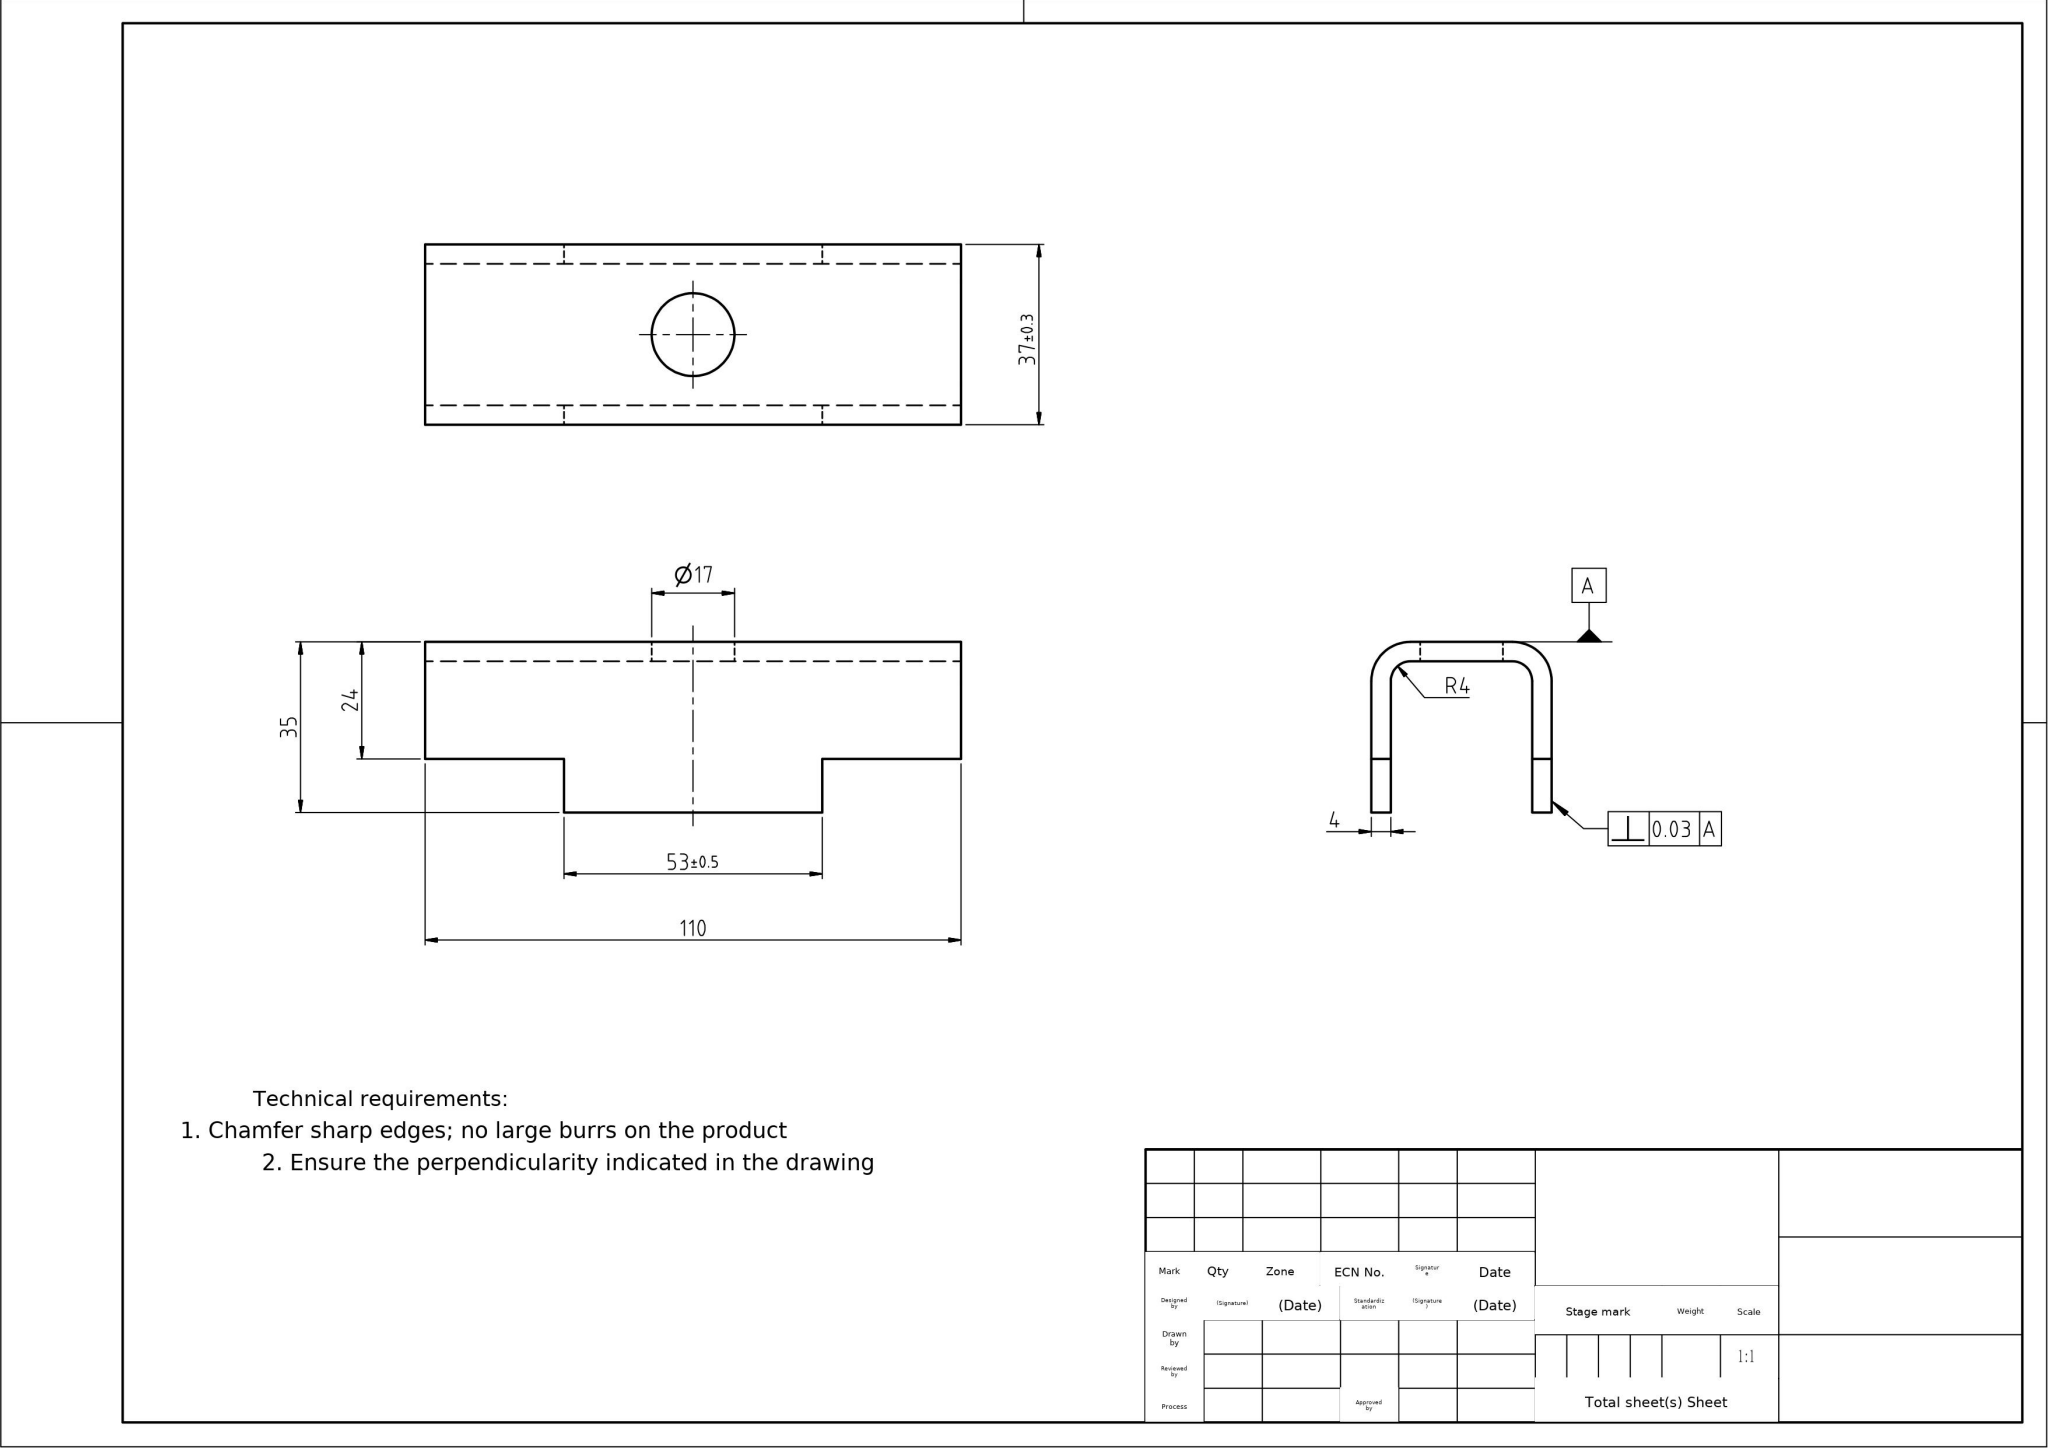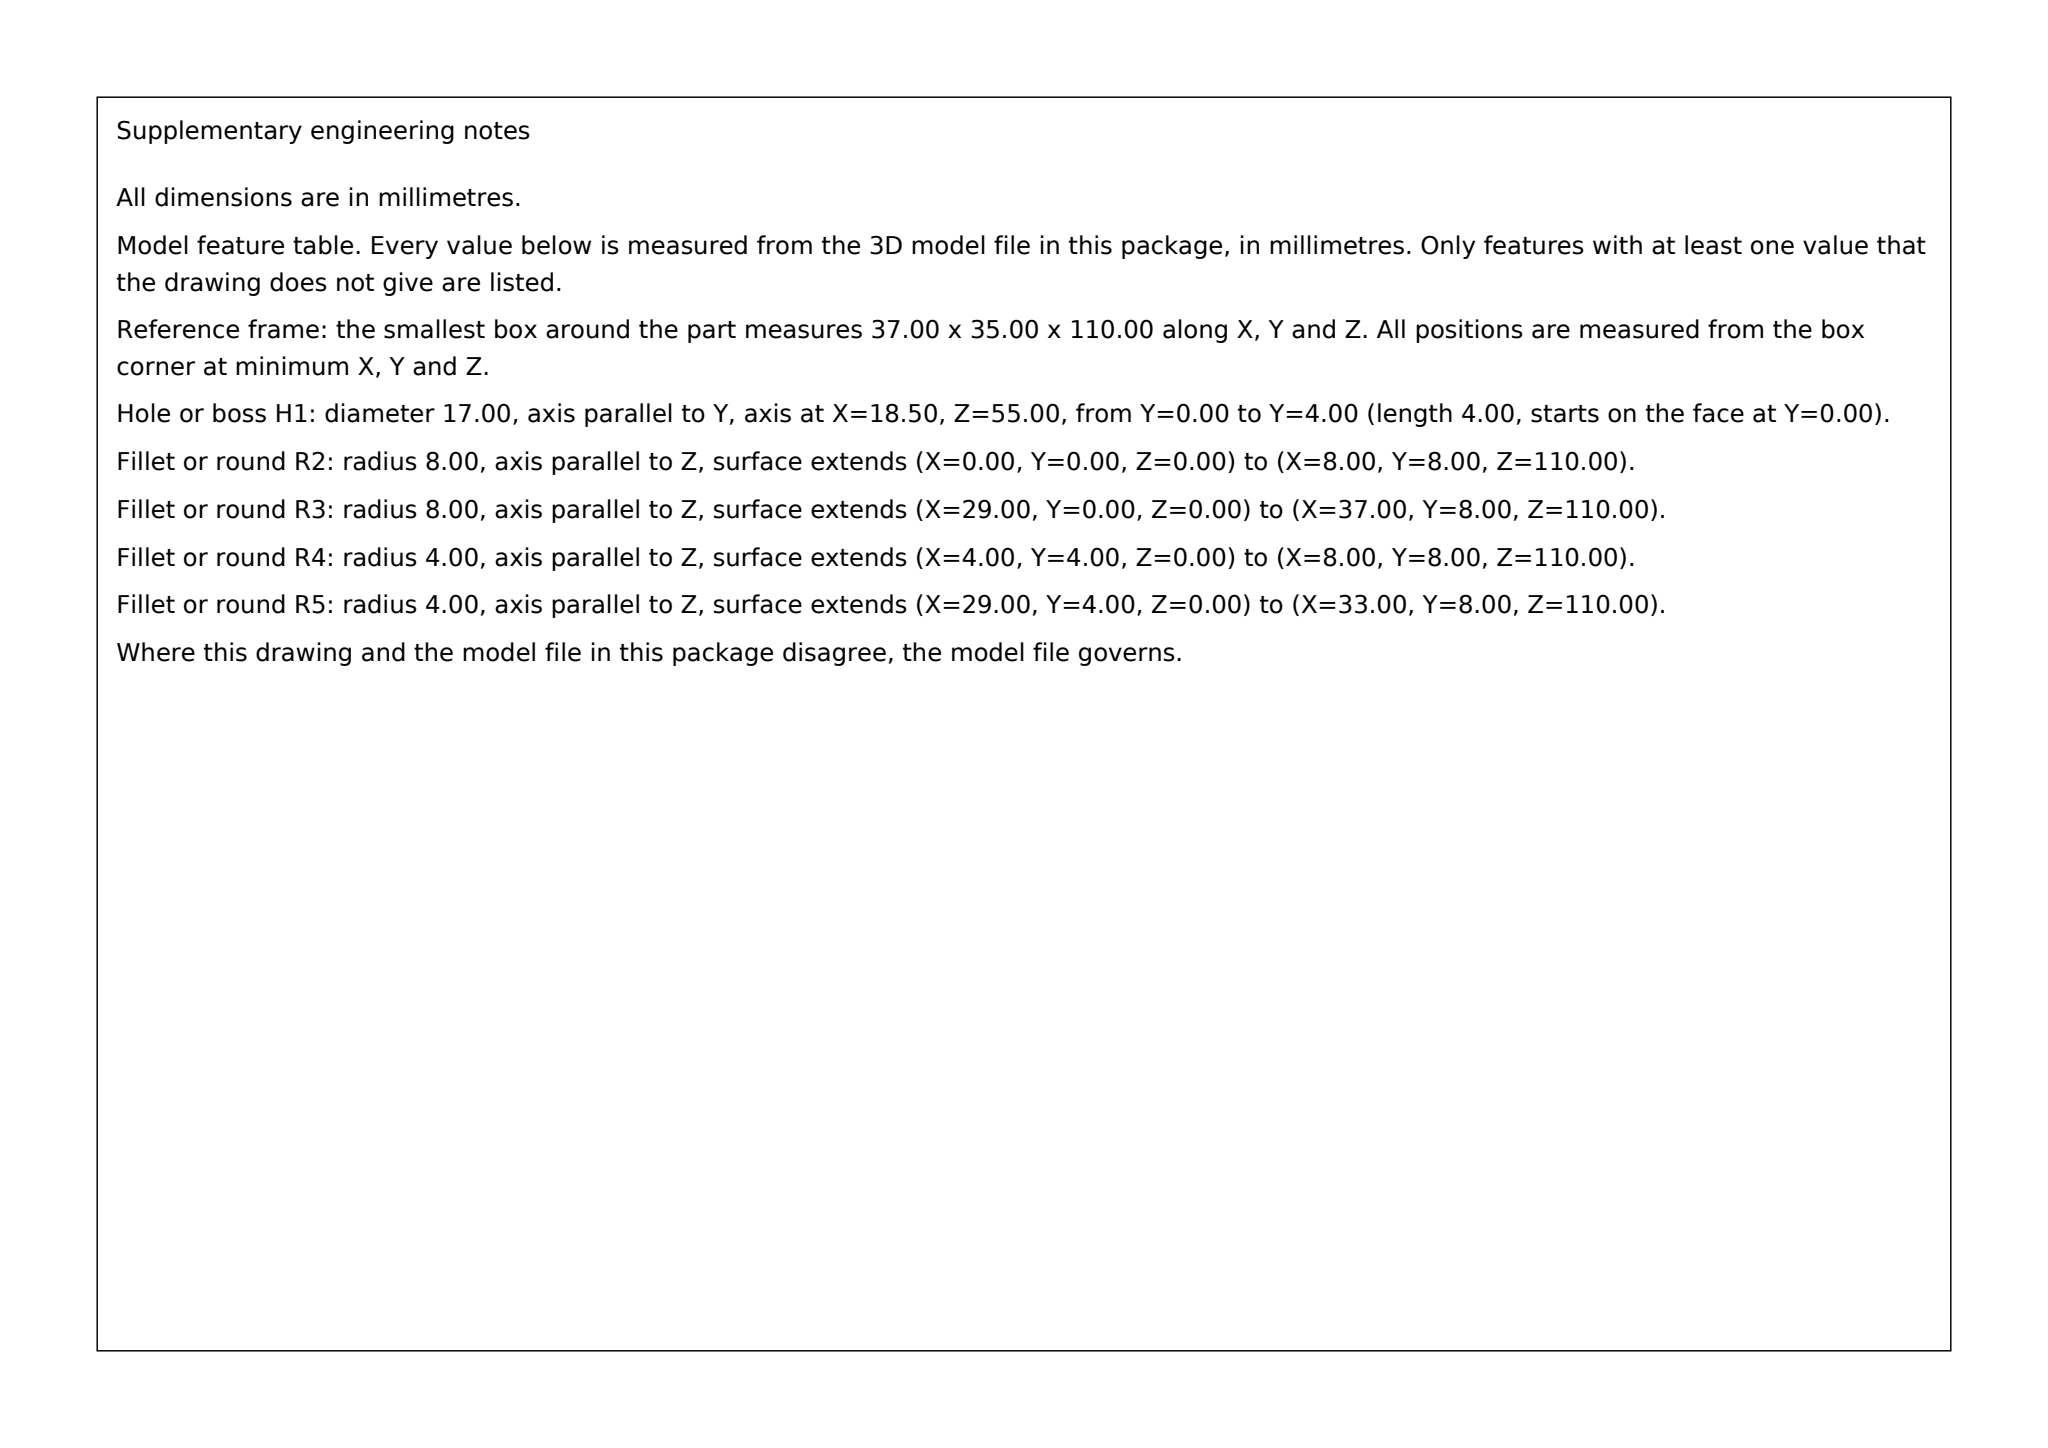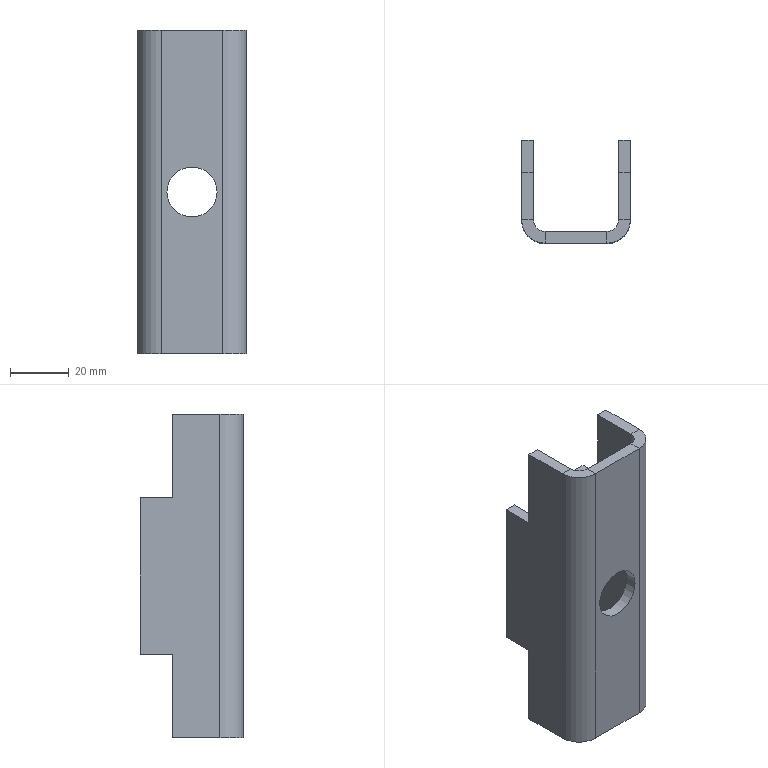Part | SolidWorks | mm | 1 solid | 32 faces | box 37 x 35 x 110 mm | volume 35370 mm3 | plane 26 | cylinder 6 | commonest cylinder face diameters 17 x2 16 x2 8 x2
STEP:
#1=CARTESIAN_POINT('',(-8.5,0.,-0.));
#2=VERTEX_POINT('',#1);
#3=CARTESIAN_POINT('',(8.5,0.,0.));
#4=VERTEX_POINT('',#3);
#5=CARTESIAN_POINT('',(0.,0.,0.));
#6=DIRECTION('',(0.,1.,0.));
#7=DIRECTION('',(1.,0.,0.));
#8=AXIS2_PLACEMENT_3D('',#5,#6,#7);
#9=CIRCLE('',#8,8.5);
#10=EDGE_CURVE('',#2,#4,#9,.T.);
#11=ORIENTED_EDGE('',*,*,#10,.F.);
#12=CARTESIAN_POINT('',(-8.5,4.,-0.));
#13=VERTEX_POINT('',#12);
#14=CARTESIAN_POINT('',(-8.5,0.,-0.));
#15=DIRECTION('',(0.,1.,0.));
#16=VECTOR('',#15,1000.);
#17=LINE('',#14,#16);
#18=EDGE_CURVE('',#2,#13,#17,.T.);
#19=ORIENTED_EDGE('',*,*,#18,.T.);
#20=CARTESIAN_POINT('',(8.5,4.,0.));
#21=VERTEX_POINT('',#20);
#22=CARTESIAN_POINT('',(0.,4.,0.));
#23=DIRECTION('',(0.,-1.,0.));
#24=DIRECTION('',(1.,0.,0.));
#25=AXIS2_PLACEMENT_3D('',#22,#23,#24);
#26=CIRCLE('',#25,8.5);
#27=EDGE_CURVE('',#21,#13,#26,.T.);
#28=ORIENTED_EDGE('',*,*,#27,.F.);
#29=CARTESIAN_POINT('',(8.5,0.,0.));
#30=DIRECTION('',(0.,1.,0.));
#31=VECTOR('',#30,1000.);
#32=LINE('',#29,#31);
#33=EDGE_CURVE('',#4,#21,#32,.T.);
#34=ORIENTED_EDGE('',*,*,#33,.F.);
#35=EDGE_LOOP('',(#11,#19,#28,#34));
#36=FACE_OUTER_BOUND('',#35,.T.);
#37=CARTESIAN_POINT('',(0.,0.,0.));
#38=DIRECTION('',(0.,1.,0.));
#39=DIRECTION('',(1.,0.,0.));
#40=AXIS2_PLACEMENT_3D('',#37,#38,#39);
#41=CYLINDRICAL_SURFACE('',#40,8.5);
#42=ADVANCED_FACE('',(#36),#41,.F.);
#43=CARTESIAN_POINT('',(18.5,35.,-26.5));
#44=VERTEX_POINT('',#43);
#45=CARTESIAN_POINT('',(14.5,35.,-26.5));
#46=VERTEX_POINT('',#45);
#47=CARTESIAN_POINT('',(16.5,35.,-26.5));
#48=DIRECTION('',(-1.,0.,-0.));
#49=VECTOR('',#48,1000.);
#50=LINE('',#47,#49);
#51=EDGE_CURVE('',#44,#46,#50,.T.);
#52=ORIENTED_EDGE('',*,*,#51,.F.);
#53=CARTESIAN_POINT('',(18.5,24.,-26.5));
#54=VERTEX_POINT('',#53);
#55=CARTESIAN_POINT('',(18.5,20.488,-26.5));
#56=DIRECTION('',(0.,1.,0.));
#57=VECTOR('',#56,1000.);
#58=LINE('',#55,#57);
#59=EDGE_CURVE('',#54,#44,#58,.T.);
#60=ORIENTED_EDGE('',*,*,#59,.F.);
#61=CARTESIAN_POINT('',(14.5,24.,-26.5));
#62=VERTEX_POINT('',#61);
#63=CARTESIAN_POINT('',(18.5,24.,-26.5));
#64=DIRECTION('',(-1.,0.,0.));
#65=VECTOR('',#64,1000.);
#66=LINE('',#63,#65);
#67=EDGE_CURVE('',#54,#62,#66,.T.);
#68=ORIENTED_EDGE('',*,*,#67,.T.);
#69=CARTESIAN_POINT('',(14.5,20.488,-26.5));
#70=DIRECTION('',(-0.,-1.,-0.));
#71=VECTOR('',#70,1000.);
#72=LINE('',#69,#71);
#73=EDGE_CURVE('',#46,#62,#72,.T.);
#74=ORIENTED_EDGE('',*,*,#73,.F.);
#75=EDGE_LOOP('',(#52,#60,#68,#74));
#76=FACE_OUTER_BOUND('',#75,.T.);
#77=CARTESIAN_POINT('',(18.5,24.,-26.5));
#78=DIRECTION('',(0.,-0.,1.));
#79=DIRECTION('',(1.,0.,0.));
#80=AXIS2_PLACEMENT_3D('',#77,#78,#79);
#81=PLANE('',#80);
#82=ADVANCED_FACE('',(#76),#81,.F.);
#83=CARTESIAN_POINT('',(14.5,24.,-55.));
#84=VERTEX_POINT('',#83);
#85=CARTESIAN_POINT('',(14.5,24.,-33.902));
#86=DIRECTION('',(0.,0.,-1.));
#87=VECTOR('',#86,1000.);
#88=LINE('',#85,#87);
#89=EDGE_CURVE('',#62,#84,#88,.T.);
#90=ORIENTED_EDGE('',*,*,#89,.F.);
#91=ORIENTED_EDGE('',*,*,#67,.F.);
#92=CARTESIAN_POINT('',(18.5,24.,-55.));
#93=VERTEX_POINT('',#92);
#94=CARTESIAN_POINT('',(18.5,24.,-33.902));
#95=DIRECTION('',(0.,-0.,1.));
#96=VECTOR('',#95,1000.);
#97=LINE('',#94,#96);
#98=EDGE_CURVE('',#93,#54,#97,.T.);
#99=ORIENTED_EDGE('',*,*,#98,.F.);
#100=CARTESIAN_POINT('',(16.5,24.,-55.));
#101=DIRECTION('',(1.,-0.,0.));
#102=VECTOR('',#101,1000.);
#103=LINE('',#100,#102);
#104=EDGE_CURVE('',#84,#93,#103,.T.);
#105=ORIENTED_EDGE('',*,*,#104,.F.);
#106=EDGE_LOOP('',(#90,#91,#99,#105));
#107=FACE_OUTER_BOUND('',#106,.T.);
#108=CARTESIAN_POINT('',(18.5,24.,-67.804));
#109=DIRECTION('',(-0.,-1.,-0.));
#110=DIRECTION('',(-1.,0.,0.));
#111=AXIS2_PLACEMENT_3D('',#108,#109,#110);
#112=PLANE('',#111);
#113=ADVANCED_FACE('',(#107),#112,.F.);
#114=CARTESIAN_POINT('',(-18.5,24.,-26.5));
#115=VERTEX_POINT('',#114);
#116=CARTESIAN_POINT('',(-18.5,24.,-55.));
#117=VERTEX_POINT('',#116);
#118=CARTESIAN_POINT('',(-18.5,24.,-33.902));
#119=DIRECTION('',(-0.,0.,-1.));
#120=VECTOR('',#119,1000.);
#121=LINE('',#118,#120);
#122=EDGE_CURVE('',#115,#117,#121,.T.);
#123=ORIENTED_EDGE('',*,*,#122,.F.);
#124=CARTESIAN_POINT('',(-14.5,24.,-26.5));
#125=VERTEX_POINT('',#124);
#126=CARTESIAN_POINT('',(18.5,24.,-26.5));
#127=DIRECTION('',(-1.,0.,0.));
#128=VECTOR('',#127,1000.);
#129=LINE('',#126,#128);
#130=EDGE_CURVE('',#125,#115,#129,.T.);
#131=ORIENTED_EDGE('',*,*,#130,.F.);
#132=CARTESIAN_POINT('',(-14.5,24.,-55.));
#133=VERTEX_POINT('',#132);
#134=CARTESIAN_POINT('',(-14.5,24.,-33.902));
#135=DIRECTION('',(0.,-0.,1.));
#136=VECTOR('',#135,1000.);
#137=LINE('',#134,#136);
#138=EDGE_CURVE('',#133,#125,#137,.T.);
#139=ORIENTED_EDGE('',*,*,#138,.F.);
#140=CARTESIAN_POINT('',(2.,24.,-55.));
#141=DIRECTION('',(1.,-0.,-0.));
#142=VECTOR('',#141,1000.);
#143=LINE('',#140,#142);
#144=EDGE_CURVE('',#117,#133,#143,.T.);
#145=ORIENTED_EDGE('',*,*,#144,.F.);
#146=EDGE_LOOP('',(#123,#131,#139,#145));
#147=FACE_OUTER_BOUND('',#146,.T.);
#148=CARTESIAN_POINT('',(18.5,24.,-67.804));
#149=DIRECTION('',(-0.,-1.,-0.));
#150=DIRECTION('',(-1.,0.,0.));
#151=AXIS2_PLACEMENT_3D('',#148,#149,#150);
#152=PLANE('',#151);
#153=ADVANCED_FACE('',(#147),#152,.F.);
#154=CARTESIAN_POINT('',(-18.5,35.,-26.5));
#155=VERTEX_POINT('',#154);
#156=CARTESIAN_POINT('',(-18.5,20.488,-26.5));
#157=DIRECTION('',(0.,-1.,-0.));
#158=VECTOR('',#157,1000.);
#159=LINE('',#156,#158);
#160=EDGE_CURVE('',#155,#115,#159,.T.);
#161=ORIENTED_EDGE('',*,*,#160,.F.);
#162=CARTESIAN_POINT('',(-14.5,35.,-26.5));
#163=VERTEX_POINT('',#162);
#164=CARTESIAN_POINT('',(2.,35.,-26.5));
#165=DIRECTION('',(-1.,-0.,-0.));
#166=VECTOR('',#165,1000.);
#167=LINE('',#164,#166);
#168=EDGE_CURVE('',#163,#155,#167,.T.);
#169=ORIENTED_EDGE('',*,*,#168,.F.);
#170=CARTESIAN_POINT('',(-14.5,20.488,-26.5));
#171=DIRECTION('',(-0.,1.,0.));
#172=VECTOR('',#171,1000.);
#173=LINE('',#170,#172);
#174=EDGE_CURVE('',#125,#163,#173,.T.);
#175=ORIENTED_EDGE('',*,*,#174,.F.);
#176=ORIENTED_EDGE('',*,*,#130,.T.);
#177=EDGE_LOOP('',(#161,#169,#175,#176));
#178=FACE_OUTER_BOUND('',#177,.T.);
#179=CARTESIAN_POINT('',(18.5,24.,-26.5));
#180=DIRECTION('',(0.,-0.,1.));
#181=DIRECTION('',(1.,0.,0.));
#182=AXIS2_PLACEMENT_3D('',#179,#180,#181);
#183=PLANE('',#182);
#184=ADVANCED_FACE('',(#178),#183,.F.);
#185=CARTESIAN_POINT('',(-18.5,24.,26.5));
#186=VERTEX_POINT('',#185);
#187=CARTESIAN_POINT('',(-18.5,35.,26.5));
#188=VERTEX_POINT('',#187);
#189=CARTESIAN_POINT('',(-18.5,30.405,26.5));
#190=DIRECTION('',(-0.,1.,0.));
#191=VECTOR('',#190,1000.);
#192=LINE('',#189,#191);
#193=EDGE_CURVE('',#186,#188,#192,.T.);
#194=ORIENTED_EDGE('',*,*,#193,.F.);
#195=CARTESIAN_POINT('',(-14.5,24.,26.5));
#196=VERTEX_POINT('',#195);
#197=CARTESIAN_POINT('',(18.5,24.,26.5));
#198=DIRECTION('',(-1.,0.,0.));
#199=VECTOR('',#198,1000.);
#200=LINE('',#197,#199);
#201=EDGE_CURVE('',#196,#186,#200,.T.);
#202=ORIENTED_EDGE('',*,*,#201,.F.);
#203=CARTESIAN_POINT('',(-14.5,35.,26.5));
#204=VERTEX_POINT('',#203);
#205=CARTESIAN_POINT('',(-14.5,30.405,26.5));
#206=DIRECTION('',(0.,-1.,0.));
#207=VECTOR('',#206,1000.);
#208=LINE('',#205,#207);
#209=EDGE_CURVE('',#204,#196,#208,.T.);
#210=ORIENTED_EDGE('',*,*,#209,.F.);
#211=CARTESIAN_POINT('',(2.,35.,26.5));
#212=DIRECTION('',(1.,0.,0.));
#213=VECTOR('',#212,1000.);
#214=LINE('',#211,#213);
#215=EDGE_CURVE('',#188,#204,#214,.T.);
#216=ORIENTED_EDGE('',*,*,#215,.F.);
#217=EDGE_LOOP('',(#194,#202,#210,#216));
#218=FACE_OUTER_BOUND('',#217,.T.);
#219=CARTESIAN_POINT('',(18.5,43.834,26.5));
#220=DIRECTION('',(0.,0.,-1.));
#221=DIRECTION('',(0.,-1.,0.));
#222=AXIS2_PLACEMENT_3D('',#219,#220,#221);
#223=PLANE('',#222);
#224=ADVANCED_FACE('',(#218),#223,.F.);
#225=CARTESIAN_POINT('',(-18.5,24.,55.));
#226=VERTEX_POINT('',#225);
#227=CARTESIAN_POINT('',(-18.5,24.,13.25));
#228=DIRECTION('',(-0.,0.,-1.));
#229=VECTOR('',#228,1000.);
#230=LINE('',#227,#229);
#231=EDGE_CURVE('',#226,#186,#230,.T.);
#232=ORIENTED_EDGE('',*,*,#231,.F.);
#233=CARTESIAN_POINT('',(-14.5,24.,55.));
#234=VERTEX_POINT('',#233);
#235=CARTESIAN_POINT('',(2.,24.,55.));
#236=DIRECTION('',(-1.,0.,0.));
#237=VECTOR('',#236,1000.);
#238=LINE('',#235,#237);
#239=EDGE_CURVE('',#234,#226,#238,.T.);
#240=ORIENTED_EDGE('',*,*,#239,.F.);
#241=CARTESIAN_POINT('',(-14.5,24.,13.25));
#242=DIRECTION('',(0.,-0.,1.));
#243=VECTOR('',#242,1000.);
#244=LINE('',#241,#243);
#245=EDGE_CURVE('',#196,#234,#244,.T.);
#246=ORIENTED_EDGE('',*,*,#245,.F.);
#247=ORIENTED_EDGE('',*,*,#201,.T.);
#248=EDGE_LOOP('',(#232,#240,#246,#247));
#249=FACE_OUTER_BOUND('',#248,.T.);
#250=CARTESIAN_POINT('',(18.5,24.,26.5));
#251=DIRECTION('',(-0.,-1.,-0.));
#252=DIRECTION('',(-1.,0.,0.));
#253=AXIS2_PLACEMENT_3D('',#250,#251,#252);
#254=PLANE('',#253);
#255=ADVANCED_FACE('',(#249),#254,.F.);
#256=CARTESIAN_POINT('',(18.5,24.,55.));
#257=VERTEX_POINT('',#256);
#258=CARTESIAN_POINT('',(14.5,24.,55.));
#259=VERTEX_POINT('',#258);
#260=CARTESIAN_POINT('',(16.5,24.,55.));
#261=DIRECTION('',(-1.,0.,0.));
#262=VECTOR('',#261,1000.);
#263=LINE('',#260,#262);
#264=EDGE_CURVE('',#257,#259,#263,.T.);
#265=ORIENTED_EDGE('',*,*,#264,.F.);
#266=CARTESIAN_POINT('',(18.5,24.,26.5));
#267=VERTEX_POINT('',#266);
#268=CARTESIAN_POINT('',(18.5,24.,13.25));
#269=DIRECTION('',(0.,-0.,1.));
#270=VECTOR('',#269,1000.);
#271=LINE('',#268,#270);
#272=EDGE_CURVE('',#267,#257,#271,.T.);
#273=ORIENTED_EDGE('',*,*,#272,.F.);
#274=CARTESIAN_POINT('',(14.5,24.,26.5));
#275=VERTEX_POINT('',#274);
#276=CARTESIAN_POINT('',(18.5,24.,26.5));
#277=DIRECTION('',(-1.,0.,0.));
#278=VECTOR('',#277,1000.);
#279=LINE('',#276,#278);
#280=EDGE_CURVE('',#267,#275,#279,.T.);
#281=ORIENTED_EDGE('',*,*,#280,.T.);
#282=CARTESIAN_POINT('',(14.5,24.,13.25));
#283=DIRECTION('',(0.,0.,-1.));
#284=VECTOR('',#283,1000.);
#285=LINE('',#282,#284);
#286=EDGE_CURVE('',#259,#275,#285,.T.);
#287=ORIENTED_EDGE('',*,*,#286,.F.);
#288=EDGE_LOOP('',(#265,#273,#281,#287));
#289=FACE_OUTER_BOUND('',#288,.T.);
#290=CARTESIAN_POINT('',(18.5,24.,26.5));
#291=DIRECTION('',(-0.,-1.,-0.));
#292=DIRECTION('',(-1.,0.,0.));
#293=AXIS2_PLACEMENT_3D('',#290,#291,#292);
#294=PLANE('',#293);
#295=ADVANCED_FACE('',(#289),#294,.F.);
#296=CARTESIAN_POINT('',(14.5,35.,26.5));
#297=VERTEX_POINT('',#296);
#298=CARTESIAN_POINT('',(18.5,35.,26.5));
#299=VERTEX_POINT('',#298);
#300=CARTESIAN_POINT('',(16.5,35.,26.5));
#301=DIRECTION('',(1.,-0.,0.));
#302=VECTOR('',#301,1000.);
#303=LINE('',#300,#302);
#304=EDGE_CURVE('',#297,#299,#303,.T.);
#305=ORIENTED_EDGE('',*,*,#304,.F.);
#306=CARTESIAN_POINT('',(14.5,30.405,26.5));
#307=DIRECTION('',(0.,1.,0.));
#308=VECTOR('',#307,1000.);
#309=LINE('',#306,#308);
#310=EDGE_CURVE('',#275,#297,#309,.T.);
#311=ORIENTED_EDGE('',*,*,#310,.F.);
#312=ORIENTED_EDGE('',*,*,#280,.F.);
#313=CARTESIAN_POINT('',(18.5,30.405,26.5));
#314=DIRECTION('',(-0.,-1.,0.));
#315=VECTOR('',#314,1000.);
#316=LINE('',#313,#315);
#317=EDGE_CURVE('',#299,#267,#316,.T.);
#318=ORIENTED_EDGE('',*,*,#317,.F.);
#319=EDGE_LOOP('',(#305,#311,#312,#318));
#320=FACE_OUTER_BOUND('',#319,.T.);
#321=CARTESIAN_POINT('',(18.5,43.834,26.5));
#322=DIRECTION('',(0.,0.,-1.));
#323=DIRECTION('',(0.,-1.,0.));
#324=AXIS2_PLACEMENT_3D('',#321,#322,#323);
#325=PLANE('',#324);
#326=ADVANCED_FACE('',(#320),#325,.F.);
#327=ORIENTED_EDGE('',*,*,#144,.T.);
#328=CARTESIAN_POINT('',(-14.5,8.,-55.));
#329=VERTEX_POINT('',#328);
#330=CARTESIAN_POINT('',(-14.5,-1.048,-55.));
#331=DIRECTION('',(-0.,1.,-0.));
#332=VECTOR('',#331,1000.);
#333=LINE('',#330,#332);
#334=EDGE_CURVE('',#329,#133,#333,.T.);
#335=ORIENTED_EDGE('',*,*,#334,.F.);
#336=CARTESIAN_POINT('',(-18.5,8.,-55.));
#337=VERTEX_POINT('',#336);
#338=CARTESIAN_POINT('',(-15.38,8.,-55.));
#339=DIRECTION('',(-1.,-0.,0.));
#340=VECTOR('',#339,1000.);
#341=LINE('',#338,#340);
#342=EDGE_CURVE('',#329,#337,#341,.T.);
#343=ORIENTED_EDGE('',*,*,#342,.T.);
#344=CARTESIAN_POINT('',(-18.5,8.,-55.));
#345=DIRECTION('',(-0.,1.,0.));
#346=VECTOR('',#345,1000.);
#347=LINE('',#344,#346);
#348=EDGE_CURVE('',#337,#117,#347,.T.);
#349=ORIENTED_EDGE('',*,*,#348,.T.);
#350=EDGE_LOOP('',(#327,#335,#343,#349));
#351=FACE_OUTER_BOUND('',#350,.T.);
#352=CARTESIAN_POINT('',(-14.5,8.,-55.));
#353=DIRECTION('',(-0.,-0.,-1.));
#354=DIRECTION('',(-1.,0.,0.));
#355=AXIS2_PLACEMENT_3D('',#352,#353,#354);
#356=PLANE('',#355);
#357=ADVANCED_FACE('',(#351),#356,.T.);
#358=ORIENTED_EDGE('',*,*,#264,.T.);
#359=CARTESIAN_POINT('',(14.5,8.,55.));
#360=VERTEX_POINT('',#359);
#361=CARTESIAN_POINT('',(14.5,-1.048,55.));
#362=DIRECTION('',(0.,1.,0.));
#363=VECTOR('',#362,1000.);
#364=LINE('',#361,#363);
#365=EDGE_CURVE('',#360,#259,#364,.T.);
#366=ORIENTED_EDGE('',*,*,#365,.F.);
#367=CARTESIAN_POINT('',(18.5,8.,55.));
#368=VERTEX_POINT('',#367);
#369=CARTESIAN_POINT('',(15.38,8.,55.));
#370=DIRECTION('',(1.,-0.,0.));
#371=VECTOR('',#370,1000.);
#372=LINE('',#369,#371);
#373=EDGE_CURVE('',#360,#368,#372,.T.);
#374=ORIENTED_EDGE('',*,*,#373,.T.);
#375=CARTESIAN_POINT('',(18.5,8.,55.));
#376=DIRECTION('',(0.,1.,0.));
#377=VECTOR('',#376,1000.);
#378=LINE('',#375,#377);
#379=EDGE_CURVE('',#368,#257,#378,.T.);
#380=ORIENTED_EDGE('',*,*,#379,.T.);
#381=EDGE_LOOP('',(#358,#366,#374,#380));
#382=FACE_OUTER_BOUND('',#381,.T.);
#383=CARTESIAN_POINT('',(14.5,8.,55.));
#384=DIRECTION('',(0.,0.,1.));
#385=DIRECTION('',(1.,0.,0.));
#386=AXIS2_PLACEMENT_3D('',#383,#384,#385);
#387=PLANE('',#386);
#388=ADVANCED_FACE('',(#382),#387,.T.);
#389=ORIENTED_EDGE('',*,*,#51,.T.);
#390=CARTESIAN_POINT('',(14.5,35.,55.));
#391=DIRECTION('',(0.,0.,-1.));
#392=VECTOR('',#391,1000.);
#393=LINE('',#390,#392);
#394=EDGE_CURVE('',#297,#46,#393,.T.);
#395=ORIENTED_EDGE('',*,*,#394,.F.);
#396=ORIENTED_EDGE('',*,*,#304,.T.);
#397=CARTESIAN_POINT('',(18.5,35.,55.));
#398=DIRECTION('',(0.,0.,-1.));
#399=VECTOR('',#398,1000.);
#400=LINE('',#397,#399);
#401=EDGE_CURVE('',#299,#44,#400,.T.);
#402=ORIENTED_EDGE('',*,*,#401,.T.);
#403=EDGE_LOOP('',(#389,#395,#396,#402));
#404=FACE_OUTER_BOUND('',#403,.T.);
#405=CARTESIAN_POINT('',(14.5,35.,55.));
#406=DIRECTION('',(0.,1.,0.));
#407=DIRECTION('',(1.,0.,-0.));
#408=AXIS2_PLACEMENT_3D('',#405,#406,#407);
#409=PLANE('',#408);
#410=ADVANCED_FACE('',(#404),#409,.T.);
#411=ORIENTED_EDGE('',*,*,#73,.T.);
#412=ORIENTED_EDGE('',*,*,#89,.T.);
#413=CARTESIAN_POINT('',(14.5,8.,-55.));
#414=VERTEX_POINT('',#413);
#415=CARTESIAN_POINT('',(14.5,-1.048,-55.));
#416=DIRECTION('',(0.,1.,0.));
#417=VECTOR('',#416,1000.);
#418=LINE('',#415,#417);
#419=EDGE_CURVE('',#414,#84,#418,.T.);
#420=ORIENTED_EDGE('',*,*,#419,.F.);
#421=CARTESIAN_POINT('',(14.5,8.,-0.));
#422=DIRECTION('',(-0.,0.,1.));
#423=VECTOR('',#422,1000.);
#424=LINE('',#421,#423);
#425=EDGE_CURVE('',#414,#360,#424,.T.);
#426=ORIENTED_EDGE('',*,*,#425,.T.);
#427=ORIENTED_EDGE('',*,*,#365,.T.);
#428=ORIENTED_EDGE('',*,*,#286,.T.);
#429=ORIENTED_EDGE('',*,*,#310,.T.);
#430=ORIENTED_EDGE('',*,*,#394,.T.);
#431=EDGE_LOOP('',(#411,#412,#420,#426,#427,#428,#429,#430));
#432=FACE_OUTER_BOUND('',#431,.T.);
#433=CARTESIAN_POINT('',(14.5,16.976,-0.));
#434=DIRECTION('',(-1.,0.,-0.));
#435=DIRECTION('',(-0.,0.,1.));
#436=AXIS2_PLACEMENT_3D('',#433,#434,#435);
#437=PLANE('',#436);
#438=ADVANCED_FACE('',(#432),#437,.T.);
#439=ORIENTED_EDGE('',*,*,#138,.T.);
#440=ORIENTED_EDGE('',*,*,#174,.T.);
#441=CARTESIAN_POINT('',(-14.5,35.,-55.));
#442=DIRECTION('',(0.,-0.,1.));
#443=VECTOR('',#442,1000.);
#444=LINE('',#441,#443);
#445=EDGE_CURVE('',#163,#204,#444,.T.);
#446=ORIENTED_EDGE('',*,*,#445,.T.);
#447=ORIENTED_EDGE('',*,*,#209,.T.);
#448=ORIENTED_EDGE('',*,*,#245,.T.);
#449=CARTESIAN_POINT('',(-14.5,8.,55.));
#450=VERTEX_POINT('',#449);
#451=CARTESIAN_POINT('',(-14.5,-1.048,55.));
#452=DIRECTION('',(-0.,1.,-0.));
#453=VECTOR('',#452,1000.);
#454=LINE('',#451,#453);
#455=EDGE_CURVE('',#450,#234,#454,.T.);
#456=ORIENTED_EDGE('',*,*,#455,.F.);
#457=CARTESIAN_POINT('',(-14.5,8.,0.));
#458=DIRECTION('',(-0.,0.,-1.));
#459=VECTOR('',#458,1000.);
#460=LINE('',#457,#459);
#461=EDGE_CURVE('',#450,#329,#460,.T.);
#462=ORIENTED_EDGE('',*,*,#461,.T.);
#463=ORIENTED_EDGE('',*,*,#334,.T.);
#464=EDGE_LOOP('',(#439,#440,#446,#447,#448,#456,#462,#463));
#465=FACE_OUTER_BOUND('',#464,.T.);
#466=CARTESIAN_POINT('',(-14.5,16.976,-0.));
#467=DIRECTION('',(1.,-0.,-0.));
#468=DIRECTION('',(0.,1.,-0.));
#469=AXIS2_PLACEMENT_3D('',#466,#467,#468);
#470=PLANE('',#469);
#471=ADVANCED_FACE('',(#465),#470,.T.);
#472=ORIENTED_EDGE('',*,*,#18,.F.);
#473=CARTESIAN_POINT('',(0.,0.,0.));
#474=DIRECTION('',(0.,1.,0.));
#475=DIRECTION('',(1.,0.,0.));
#476=AXIS2_PLACEMENT_3D('',#473,#474,#475);
#477=CIRCLE('',#476,8.5);
#478=EDGE_CURVE('',#4,#2,#477,.T.);
#479=ORIENTED_EDGE('',*,*,#478,.F.);
#480=ORIENTED_EDGE('',*,*,#33,.T.);
#481=CARTESIAN_POINT('',(0.,4.,0.));
#482=DIRECTION('',(0.,-1.,0.));
#483=DIRECTION('',(1.,0.,0.));
#484=AXIS2_PLACEMENT_3D('',#481,#482,#483);
#485=CIRCLE('',#484,8.5);
#486=EDGE_CURVE('',#13,#21,#485,.T.);
#487=ORIENTED_EDGE('',*,*,#486,.F.);
#488=EDGE_LOOP('',(#472,#479,#480,#487));
#489=FACE_OUTER_BOUND('',#488,.T.);
#490=CARTESIAN_POINT('',(0.,0.,0.));
#491=DIRECTION('',(0.,1.,0.));
#492=DIRECTION('',(1.,0.,0.));
#493=AXIS2_PLACEMENT_3D('',#490,#491,#492);
#494=CYLINDRICAL_SURFACE('',#493,8.5);
#495=ADVANCED_FACE('',(#489),#494,.F.);
#496=CARTESIAN_POINT('',(-18.5,8.,55.));
#497=VERTEX_POINT('',#496);
#498=CARTESIAN_POINT('',(-18.5,8.,0.));
#499=DIRECTION('',(0.,0.,1.));
#500=VECTOR('',#499,1000.);
#501=LINE('',#498,#500);
#502=EDGE_CURVE('',#337,#497,#501,.T.);
#503=ORIENTED_EDGE('',*,*,#502,.F.);
#504=CARTESIAN_POINT('',(-10.5,-0.,-55.));
#505=VERTEX_POINT('',#504);
#506=CARTESIAN_POINT('',(-10.5,8.,-55.));
#507=DIRECTION('',(-0.,0.,-1.));
#508=DIRECTION('',(-0.,-1.,0.));
#509=AXIS2_PLACEMENT_3D('',#506,#507,#508);
#510=CIRCLE('',#509,8.);
#511=EDGE_CURVE('',#505,#337,#510,.T.);
#512=ORIENTED_EDGE('',*,*,#511,.F.);
#513=CARTESIAN_POINT('',(-10.5,-0.,55.));
#514=VERTEX_POINT('',#513);
#515=CARTESIAN_POINT('',(-10.5,0.,27.5));
#516=DIRECTION('',(-0.,0.,-1.));
#517=VECTOR('',#516,1000.);
#518=LINE('',#515,#517);
#519=EDGE_CURVE('',#514,#505,#518,.T.);
#520=ORIENTED_EDGE('',*,*,#519,.F.);
#521=CARTESIAN_POINT('',(-10.5,8.,55.));
#522=DIRECTION('',(0.,0.,1.));
#523=DIRECTION('',(-1.,0.,0.));
#524=AXIS2_PLACEMENT_3D('',#521,#522,#523);
#525=CIRCLE('',#524,8.);
#526=EDGE_CURVE('',#497,#514,#525,.T.);
#527=ORIENTED_EDGE('',*,*,#526,.F.);
#528=EDGE_LOOP('',(#503,#512,#520,#527));
#529=FACE_OUTER_BOUND('',#528,.T.);
#530=CARTESIAN_POINT('',(-10.5,8.,0.));
#531=DIRECTION('',(-0.,0.,-1.));
#532=DIRECTION('',(0.,-1.,0.));
#533=AXIS2_PLACEMENT_3D('',#530,#531,#532);
#534=CYLINDRICAL_SURFACE('',#533,8.);
#535=ADVANCED_FACE('',(#529),#534,.T.);
#536=ORIENTED_EDGE('',*,*,#239,.T.);
#537=CARTESIAN_POINT('',(-18.5,-1.048,55.));
#538=DIRECTION('',(0.,-1.,0.));
#539=VECTOR('',#538,1000.);
#540=LINE('',#537,#539);
#541=EDGE_CURVE('',#226,#497,#540,.T.);
#542=ORIENTED_EDGE('',*,*,#541,.T.);
#543=CARTESIAN_POINT('',(-15.38,8.,55.));
#544=DIRECTION('',(1.,0.,-0.));
#545=VECTOR('',#544,1000.);
#546=LINE('',#543,#545);
#547=EDGE_CURVE('',#497,#450,#546,.T.);
#548=ORIENTED_EDGE('',*,*,#547,.T.);
#549=ORIENTED_EDGE('',*,*,#455,.T.);
#550=EDGE_LOOP('',(#536,#542,#548,#549));
#551=FACE_OUTER_BOUND('',#550,.T.);
#552=CARTESIAN_POINT('',(-14.5,8.,55.));
#553=DIRECTION('',(0.,0.,1.));
#554=DIRECTION('',(1.,-0.,0.));
#555=AXIS2_PLACEMENT_3D('',#552,#553,#554);
#556=PLANE('',#555);
#557=ADVANCED_FACE('',(#551),#556,.T.);
#558=ORIENTED_EDGE('',*,*,#342,.F.);
#559=CARTESIAN_POINT('',(-10.5,4.,-55.));
#560=VERTEX_POINT('',#559);
#561=CARTESIAN_POINT('',(-10.5,8.,-55.));
#562=DIRECTION('',(-0.,0.,-1.));
#563=DIRECTION('',(0.,-1.,0.));
#564=AXIS2_PLACEMENT_3D('',#561,#562,#563);
#565=CIRCLE('',#564,4.);
#566=EDGE_CURVE('',#560,#329,#565,.T.);
#567=ORIENTED_EDGE('',*,*,#566,.F.);
#568=CARTESIAN_POINT('',(-10.5,2.,-55.));
#569=DIRECTION('',(0.,1.,0.));
#570=VECTOR('',#569,1000.);
#571=LINE('',#568,#570);
#572=EDGE_CURVE('',#505,#560,#571,.T.);
#573=ORIENTED_EDGE('',*,*,#572,.F.);
#574=ORIENTED_EDGE('',*,*,#511,.T.);
#575=EDGE_LOOP('',(#558,#567,#573,#574));
#576=FACE_OUTER_BOUND('',#575,.T.);
#577=CARTESIAN_POINT('',(-14.5,8.,-55.));
#578=DIRECTION('',(-0.,0.,-1.));
#579=DIRECTION('',(-1.,0.,0.));
#580=AXIS2_PLACEMENT_3D('',#577,#578,#579);
#581=PLANE('',#580);
#582=ADVANCED_FACE('',(#576),#581,.T.);
#583=ORIENTED_EDGE('',*,*,#547,.F.);
#584=ORIENTED_EDGE('',*,*,#526,.T.);
#585=CARTESIAN_POINT('',(-10.5,4.,55.));
#586=VERTEX_POINT('',#585);
#587=CARTESIAN_POINT('',(-10.5,2.,55.));
#588=DIRECTION('',(0.,-1.,0.));
#589=VECTOR('',#588,1000.);
#590=LINE('',#587,#589);
#591=EDGE_CURVE('',#586,#514,#590,.T.);
#592=ORIENTED_EDGE('',*,*,#591,.F.);
#593=CARTESIAN_POINT('',(-10.5,8.,55.));
#594=DIRECTION('',(-0.,0.,-1.));
#595=DIRECTION('',(0.,-1.,0.));
#596=AXIS2_PLACEMENT_3D('',#593,#594,#595);
#597=CIRCLE('',#596,4.);
#598=EDGE_CURVE('',#586,#450,#597,.T.);
#599=ORIENTED_EDGE('',*,*,#598,.T.);
#600=EDGE_LOOP('',(#583,#584,#592,#599));
#601=FACE_OUTER_BOUND('',#600,.T.);
#602=CARTESIAN_POINT('',(-18.5,8.,55.));
#603=DIRECTION('',(0.,0.,1.));
#604=DIRECTION('',(1.,-0.,0.));
#605=AXIS2_PLACEMENT_3D('',#602,#603,#604);
#606=PLANE('',#605);
#607=ADVANCED_FACE('',(#601),#606,.T.);
#608=ORIENTED_EDGE('',*,*,#168,.T.);
#609=CARTESIAN_POINT('',(-18.5,35.,-55.));
#610=DIRECTION('',(0.,-0.,1.));
#611=VECTOR('',#610,1000.);
#612=LINE('',#609,#611);
#613=EDGE_CURVE('',#155,#188,#612,.T.);
#614=ORIENTED_EDGE('',*,*,#613,.T.);
#615=ORIENTED_EDGE('',*,*,#215,.T.);
#616=ORIENTED_EDGE('',*,*,#445,.F.);
#617=EDGE_LOOP('',(#608,#614,#615,#616));
#618=FACE_OUTER_BOUND('',#617,.T.);
#619=CARTESIAN_POINT('',(-14.5,35.,-55.));
#620=DIRECTION('',(-0.,1.,0.));
#621=DIRECTION('',(1.,0.,0.));
#622=AXIS2_PLACEMENT_3D('',#619,#620,#621);
#623=PLANE('',#622);
#624=ADVANCED_FACE('',(#618),#623,.T.);
#625=ORIENTED_EDGE('',*,*,#122,.T.);
#626=ORIENTED_EDGE('',*,*,#348,.F.);
#627=ORIENTED_EDGE('',*,*,#502,.T.);
#628=ORIENTED_EDGE('',*,*,#541,.F.);
#629=ORIENTED_EDGE('',*,*,#231,.T.);
#630=ORIENTED_EDGE('',*,*,#193,.T.);
#631=ORIENTED_EDGE('',*,*,#613,.F.);
#632=ORIENTED_EDGE('',*,*,#160,.T.);
#633=EDGE_LOOP('',(#625,#626,#627,#628,#629,#630,#631,#632));
#634=FACE_OUTER_BOUND('',#633,.T.);
#635=CARTESIAN_POINT('',(-18.5,16.976,0.));
#636=DIRECTION('',(1.,-0.,-0.));
#637=DIRECTION('',(0.,1.,-0.));
#638=AXIS2_PLACEMENT_3D('',#635,#636,#637);
#639=PLANE('',#638);
#640=ADVANCED_FACE('',(#634),#639,.F.);
#641=ORIENTED_EDGE('',*,*,#461,.F.);
#642=ORIENTED_EDGE('',*,*,#598,.F.);
#643=CARTESIAN_POINT('',(-10.5,4.,27.5));
#644=DIRECTION('',(0.,0.,1.));
#645=VECTOR('',#644,1000.);
#646=LINE('',#643,#645);
#647=EDGE_CURVE('',#560,#586,#646,.T.);
#648=ORIENTED_EDGE('',*,*,#647,.F.);
#649=ORIENTED_EDGE('',*,*,#566,.T.);
#650=EDGE_LOOP('',(#641,#642,#648,#649));
#651=FACE_OUTER_BOUND('',#650,.T.);
#652=CARTESIAN_POINT('',(-10.5,8.,0.));
#653=DIRECTION('',(-0.,0.,-1.));
#654=DIRECTION('',(0.,-1.,0.));
#655=AXIS2_PLACEMENT_3D('',#652,#653,#654);
#656=CYLINDRICAL_SURFACE('',#655,4.);
#657=ADVANCED_FACE('',(#651),#656,.F.);
#658=CARTESIAN_POINT('',(18.5,8.,-55.));
#659=VERTEX_POINT('',#658);
#660=CARTESIAN_POINT('',(18.5,8.,-0.));
#661=DIRECTION('',(-0.,0.,-1.));
#662=VECTOR('',#661,1000.);
#663=LINE('',#660,#662);
#664=EDGE_CURVE('',#368,#659,#663,.T.);
#665=ORIENTED_EDGE('',*,*,#664,.F.);
#666=CARTESIAN_POINT('',(10.5,-0.,55.));
#667=VERTEX_POINT('',#666);
#668=CARTESIAN_POINT('',(10.5,8.,55.));
#669=DIRECTION('',(0.,0.,1.));
#670=DIRECTION('',(0.,-1.,0.));
#671=AXIS2_PLACEMENT_3D('',#668,#669,#670);
#672=CIRCLE('',#671,8.);
#673=EDGE_CURVE('',#667,#368,#672,.T.);
#674=ORIENTED_EDGE('',*,*,#673,.F.);
#675=CARTESIAN_POINT('',(10.5,-0.,-55.));
#676=VERTEX_POINT('',#675);
#677=CARTESIAN_POINT('',(10.5,0.,-27.5));
#678=DIRECTION('',(0.,0.,1.));
#679=VECTOR('',#678,1000.);
#680=LINE('',#677,#679);
#681=EDGE_CURVE('',#676,#667,#680,.T.);
#682=ORIENTED_EDGE('',*,*,#681,.F.);
#683=CARTESIAN_POINT('',(10.5,8.,-55.));
#684=DIRECTION('',(0.,0.,-1.));
#685=DIRECTION('',(1.,-0.,0.));
#686=AXIS2_PLACEMENT_3D('',#683,#684,#685);
#687=CIRCLE('',#686,8.);
#688=EDGE_CURVE('',#659,#676,#687,.T.);
#689=ORIENTED_EDGE('',*,*,#688,.F.);
#690=EDGE_LOOP('',(#665,#674,#682,#689));
#691=FACE_OUTER_BOUND('',#690,.T.);
#692=CARTESIAN_POINT('',(10.5,8.,0.));
#693=DIRECTION('',(0.,0.,1.));
#694=DIRECTION('',(0.,-1.,0.));
#695=AXIS2_PLACEMENT_3D('',#692,#693,#694);
#696=CYLINDRICAL_SURFACE('',#695,8.);
#697=ADVANCED_FACE('',(#691),#696,.T.);
#698=ORIENTED_EDGE('',*,*,#104,.T.);
#699=CARTESIAN_POINT('',(18.5,-1.048,-55.));
#700=DIRECTION('',(-0.,-1.,0.));
#701=VECTOR('',#700,1000.);
#702=LINE('',#699,#701);
#703=EDGE_CURVE('',#93,#659,#702,.T.);
#704=ORIENTED_EDGE('',*,*,#703,.T.);
#705=CARTESIAN_POINT('',(15.38,8.,-55.));
#706=DIRECTION('',(-1.,0.,0.));
#707=VECTOR('',#706,1000.);
#708=LINE('',#705,#707);
#709=EDGE_CURVE('',#659,#414,#708,.T.);
#710=ORIENTED_EDGE('',*,*,#709,.T.);
#711=ORIENTED_EDGE('',*,*,#419,.T.);
#712=EDGE_LOOP('',(#698,#704,#710,#711));
#713=FACE_OUTER_BOUND('',#712,.T.);
#714=CARTESIAN_POINT('',(14.5,8.,-55.));
#715=DIRECTION('',(0.,0.,-1.));
#716=DIRECTION('',(0.,-1.,0.));
#717=AXIS2_PLACEMENT_3D('',#714,#715,#716);
#718=PLANE('',#717);
#719=ADVANCED_FACE('',(#713),#718,.T.);
#720=ORIENTED_EDGE('',*,*,#373,.F.);
#721=CARTESIAN_POINT('',(10.5,4.,55.));
#722=VERTEX_POINT('',#721);
#723=CARTESIAN_POINT('',(10.5,8.,55.));
#724=DIRECTION('',(0.,0.,1.));
#725=DIRECTION('',(0.,-1.,0.));
#726=AXIS2_PLACEMENT_3D('',#723,#724,#725);
#727=CIRCLE('',#726,4.);
#728=EDGE_CURVE('',#722,#360,#727,.T.);
#729=ORIENTED_EDGE('',*,*,#728,.F.);
#730=CARTESIAN_POINT('',(10.5,2.,55.));
#731=DIRECTION('',(0.,1.,0.));
#732=VECTOR('',#731,1000.);
#733=LINE('',#730,#732);
#734=EDGE_CURVE('',#667,#722,#733,.T.);
#735=ORIENTED_EDGE('',*,*,#734,.F.);
#736=ORIENTED_EDGE('',*,*,#673,.T.);
#737=EDGE_LOOP('',(#720,#729,#735,#736));
#738=FACE_OUTER_BOUND('',#737,.T.);
#739=CARTESIAN_POINT('',(14.5,8.,55.));
#740=DIRECTION('',(0.,0.,1.));
#741=DIRECTION('',(1.,0.,0.));
#742=AXIS2_PLACEMENT_3D('',#739,#740,#741);
#743=PLANE('',#742);
#744=ADVANCED_FACE('',(#738),#743,.T.);
#745=ORIENTED_EDGE('',*,*,#709,.F.);
#746=ORIENTED_EDGE('',*,*,#688,.T.);
#747=CARTESIAN_POINT('',(10.5,4.,-55.));
#748=VERTEX_POINT('',#747);
#749=CARTESIAN_POINT('',(10.5,2.,-55.));
#750=DIRECTION('',(0.,-1.,0.));
#751=VECTOR('',#750,1000.);
#752=LINE('',#749,#751);
#753=EDGE_CURVE('',#748,#676,#752,.T.);
#754=ORIENTED_EDGE('',*,*,#753,.F.);
#755=CARTESIAN_POINT('',(10.5,8.,-55.));
#756=DIRECTION('',(0.,0.,1.));
#757=DIRECTION('',(0.,-1.,0.));
#758=AXIS2_PLACEMENT_3D('',#755,#756,#757);
#759=CIRCLE('',#758,4.);
#760=EDGE_CURVE('',#748,#414,#759,.T.);
#761=ORIENTED_EDGE('',*,*,#760,.T.);
#762=EDGE_LOOP('',(#745,#746,#754,#761));
#763=FACE_OUTER_BOUND('',#762,.T.);
#764=CARTESIAN_POINT('',(18.5,8.,-55.));
#765=DIRECTION('',(0.,0.,-1.));
#766=DIRECTION('',(0.,-1.,0.));
#767=AXIS2_PLACEMENT_3D('',#764,#765,#766);
#768=PLANE('',#767);
#769=ADVANCED_FACE('',(#763),#768,.T.);
#770=ORIENTED_EDGE('',*,*,#59,.T.);
#771=ORIENTED_EDGE('',*,*,#401,.F.);
#772=ORIENTED_EDGE('',*,*,#317,.T.);
#773=ORIENTED_EDGE('',*,*,#272,.T.);
#774=ORIENTED_EDGE('',*,*,#379,.F.);
#775=ORIENTED_EDGE('',*,*,#664,.T.);
#776=ORIENTED_EDGE('',*,*,#703,.F.);
#777=ORIENTED_EDGE('',*,*,#98,.T.);
#778=EDGE_LOOP('',(#770,#771,#772,#773,#774,#775,#776,#777));
#779=FACE_OUTER_BOUND('',#778,.T.);
#780=CARTESIAN_POINT('',(18.5,16.976,-0.));
#781=DIRECTION('',(-1.,0.,0.));
#782=DIRECTION('',(0.,0.,1.));
#783=AXIS2_PLACEMENT_3D('',#780,#781,#782);
#784=PLANE('',#783);
#785=ADVANCED_FACE('',(#779),#784,.F.);
#786=ORIENTED_EDGE('',*,*,#425,.F.);
#787=ORIENTED_EDGE('',*,*,#760,.F.);
#788=CARTESIAN_POINT('',(10.5,4.,-27.5));
#789=DIRECTION('',(0.,0.,-1.));
#790=VECTOR('',#789,1000.);
#791=LINE('',#788,#790);
#792=EDGE_CURVE('',#722,#748,#791,.T.);
#793=ORIENTED_EDGE('',*,*,#792,.F.);
#794=ORIENTED_EDGE('',*,*,#728,.T.);
#795=EDGE_LOOP('',(#786,#787,#793,#794));
#796=FACE_OUTER_BOUND('',#795,.T.);
#797=CARTESIAN_POINT('',(10.5,8.,0.));
#798=DIRECTION('',(0.,0.,1.));
#799=DIRECTION('',(0.,-1.,0.));
#800=AXIS2_PLACEMENT_3D('',#797,#798,#799);
#801=CYLINDRICAL_SURFACE('',#800,4.);
#802=ADVANCED_FACE('',(#796),#801,.F.);
#803=ORIENTED_EDGE('',*,*,#591,.T.);
#804=CARTESIAN_POINT('',(-18.5,0.,55.));
#805=DIRECTION('',(1.,0.,-0.));
#806=VECTOR('',#805,1000.);
#807=LINE('',#804,#806);
#808=EDGE_CURVE('',#514,#667,#807,.T.);
#809=ORIENTED_EDGE('',*,*,#808,.T.);
#810=ORIENTED_EDGE('',*,*,#734,.T.);
#811=CARTESIAN_POINT('',(-18.5,4.,55.));
#812=DIRECTION('',(-1.,0.,0.));
#813=VECTOR('',#812,1000.);
#814=LINE('',#811,#813);
#815=EDGE_CURVE('',#722,#586,#814,.T.);
#816=ORIENTED_EDGE('',*,*,#815,.T.);
#817=EDGE_LOOP('',(#803,#809,#810,#816));
#818=FACE_OUTER_BOUND('',#817,.T.);
#819=CARTESIAN_POINT('',(18.5,0.,55.));
#820=DIRECTION('',(0.,0.,1.));
#821=DIRECTION('',(1.,-0.,0.));
#822=AXIS2_PLACEMENT_3D('',#819,#820,#821);
#823=PLANE('',#822);
#824=ADVANCED_FACE('',(#818),#823,.T.);
#825=ORIENTED_EDGE('',*,*,#519,.T.);
#826=CARTESIAN_POINT('',(18.5,0.,-55.));
#827=DIRECTION('',(-1.,0.,0.));
#828=VECTOR('',#827,1000.);
#829=LINE('',#826,#828);
#830=EDGE_CURVE('',#676,#505,#829,.T.);
#831=ORIENTED_EDGE('',*,*,#830,.F.);
#832=ORIENTED_EDGE('',*,*,#681,.T.);
#833=ORIENTED_EDGE('',*,*,#808,.F.);
#834=EDGE_LOOP('',(#825,#831,#832,#833));
#835=FACE_OUTER_BOUND('',#834,.T.);
#836=ORIENTED_EDGE('',*,*,#478,.T.);
#837=ORIENTED_EDGE('',*,*,#10,.T.);
#838=EDGE_LOOP('',(#836,#837));
#839=FACE_BOUND('',#838,.T.);
#840=CARTESIAN_POINT('',(0.,0.,-0.));
#841=DIRECTION('',(0.,1.,0.));
#842=DIRECTION('',(1.,0.,0.));
#843=AXIS2_PLACEMENT_3D('',#840,#841,#842);
#844=PLANE('',#843);
#845=ADVANCED_FACE('',(#835,#839),#844,.F.);
#846=ORIENTED_EDGE('',*,*,#572,.T.);
#847=CARTESIAN_POINT('',(18.5,4.,-55.));
#848=DIRECTION('',(1.,0.,0.));
#849=VECTOR('',#848,1000.);
#850=LINE('',#847,#849);
#851=EDGE_CURVE('',#560,#748,#850,.T.);
#852=ORIENTED_EDGE('',*,*,#851,.T.);
#853=ORIENTED_EDGE('',*,*,#753,.T.);
#854=ORIENTED_EDGE('',*,*,#830,.T.);
#855=EDGE_LOOP('',(#846,#852,#853,#854));
#856=FACE_OUTER_BOUND('',#855,.T.);
#857=CARTESIAN_POINT('',(-18.5,0.,-55.));
#858=DIRECTION('',(0.,0.,-1.));
#859=DIRECTION('',(0.,-1.,0.));
#860=AXIS2_PLACEMENT_3D('',#857,#858,#859);
#861=PLANE('',#860);
#862=ADVANCED_FACE('',(#856),#861,.T.);
#863=ORIENTED_EDGE('',*,*,#647,.T.);
#864=ORIENTED_EDGE('',*,*,#815,.F.);
#865=ORIENTED_EDGE('',*,*,#792,.T.);
#866=ORIENTED_EDGE('',*,*,#851,.F.);
#867=EDGE_LOOP('',(#863,#864,#865,#866));
#868=FACE_OUTER_BOUND('',#867,.T.);
#869=ORIENTED_EDGE('',*,*,#27,.T.);
#870=ORIENTED_EDGE('',*,*,#486,.T.);
#871=EDGE_LOOP('',(#869,#870));
#872=FACE_BOUND('',#871,.T.);
#873=CARTESIAN_POINT('',(0.,4.,-0.));
#874=DIRECTION('',(0.,1.,0.));
#875=DIRECTION('',(1.,0.,0.));
#876=AXIS2_PLACEMENT_3D('',#873,#874,#875);
#877=PLANE('',#876);
#878=ADVANCED_FACE('',(#868,#872),#877,.T.);
#879=CLOSED_SHELL('',(#42,#82,#113,#153,#184,#224,#255,#295,#326,#357,#388,#410,#438,#471,#495,#535,#557,#582,#607,#624,#640,#657,#697,#719,#744,#769,#785,#802,#824,#845,#862,#878));
#880=MANIFOLD_SOLID_BREP('',#879);
#881=CARTESIAN_POINT('',(0.,0.,0.));
#882=DIRECTION('',(0.,0.,1.));
#883=DIRECTION('',(1.,0.,0.));
#884=AXIS2_PLACEMENT_3D('',#881,#882,#883);
#885=(LENGTH_UNIT()NAMED_UNIT(*)SI_UNIT(.MILLI.,.METRE.));
#886=UNCERTAINTY_MEASURE_WITH_UNIT(LENGTH_MEASURE(0.00001),#885,'','');
#887=(NAMED_UNIT(*)PLANE_ANGLE_UNIT()SI_UNIT($,.RADIAN.));
#888=(NAMED_UNIT(*)SI_UNIT($,.STERADIAN.)SOLID_ANGLE_UNIT());
#889=(GEOMETRIC_REPRESENTATION_CONTEXT(3)GLOBAL_UNCERTAINTY_ASSIGNED_CONTEXT((#886))GLOBAL_UNIT_ASSIGNED_CONTEXT((#885,#887,#888))REPRESENTATION_CONTEXT('',''));
#890=ADVANCED_BREP_SHAPE_REPRESENTATION('',(#880,#884),#889);